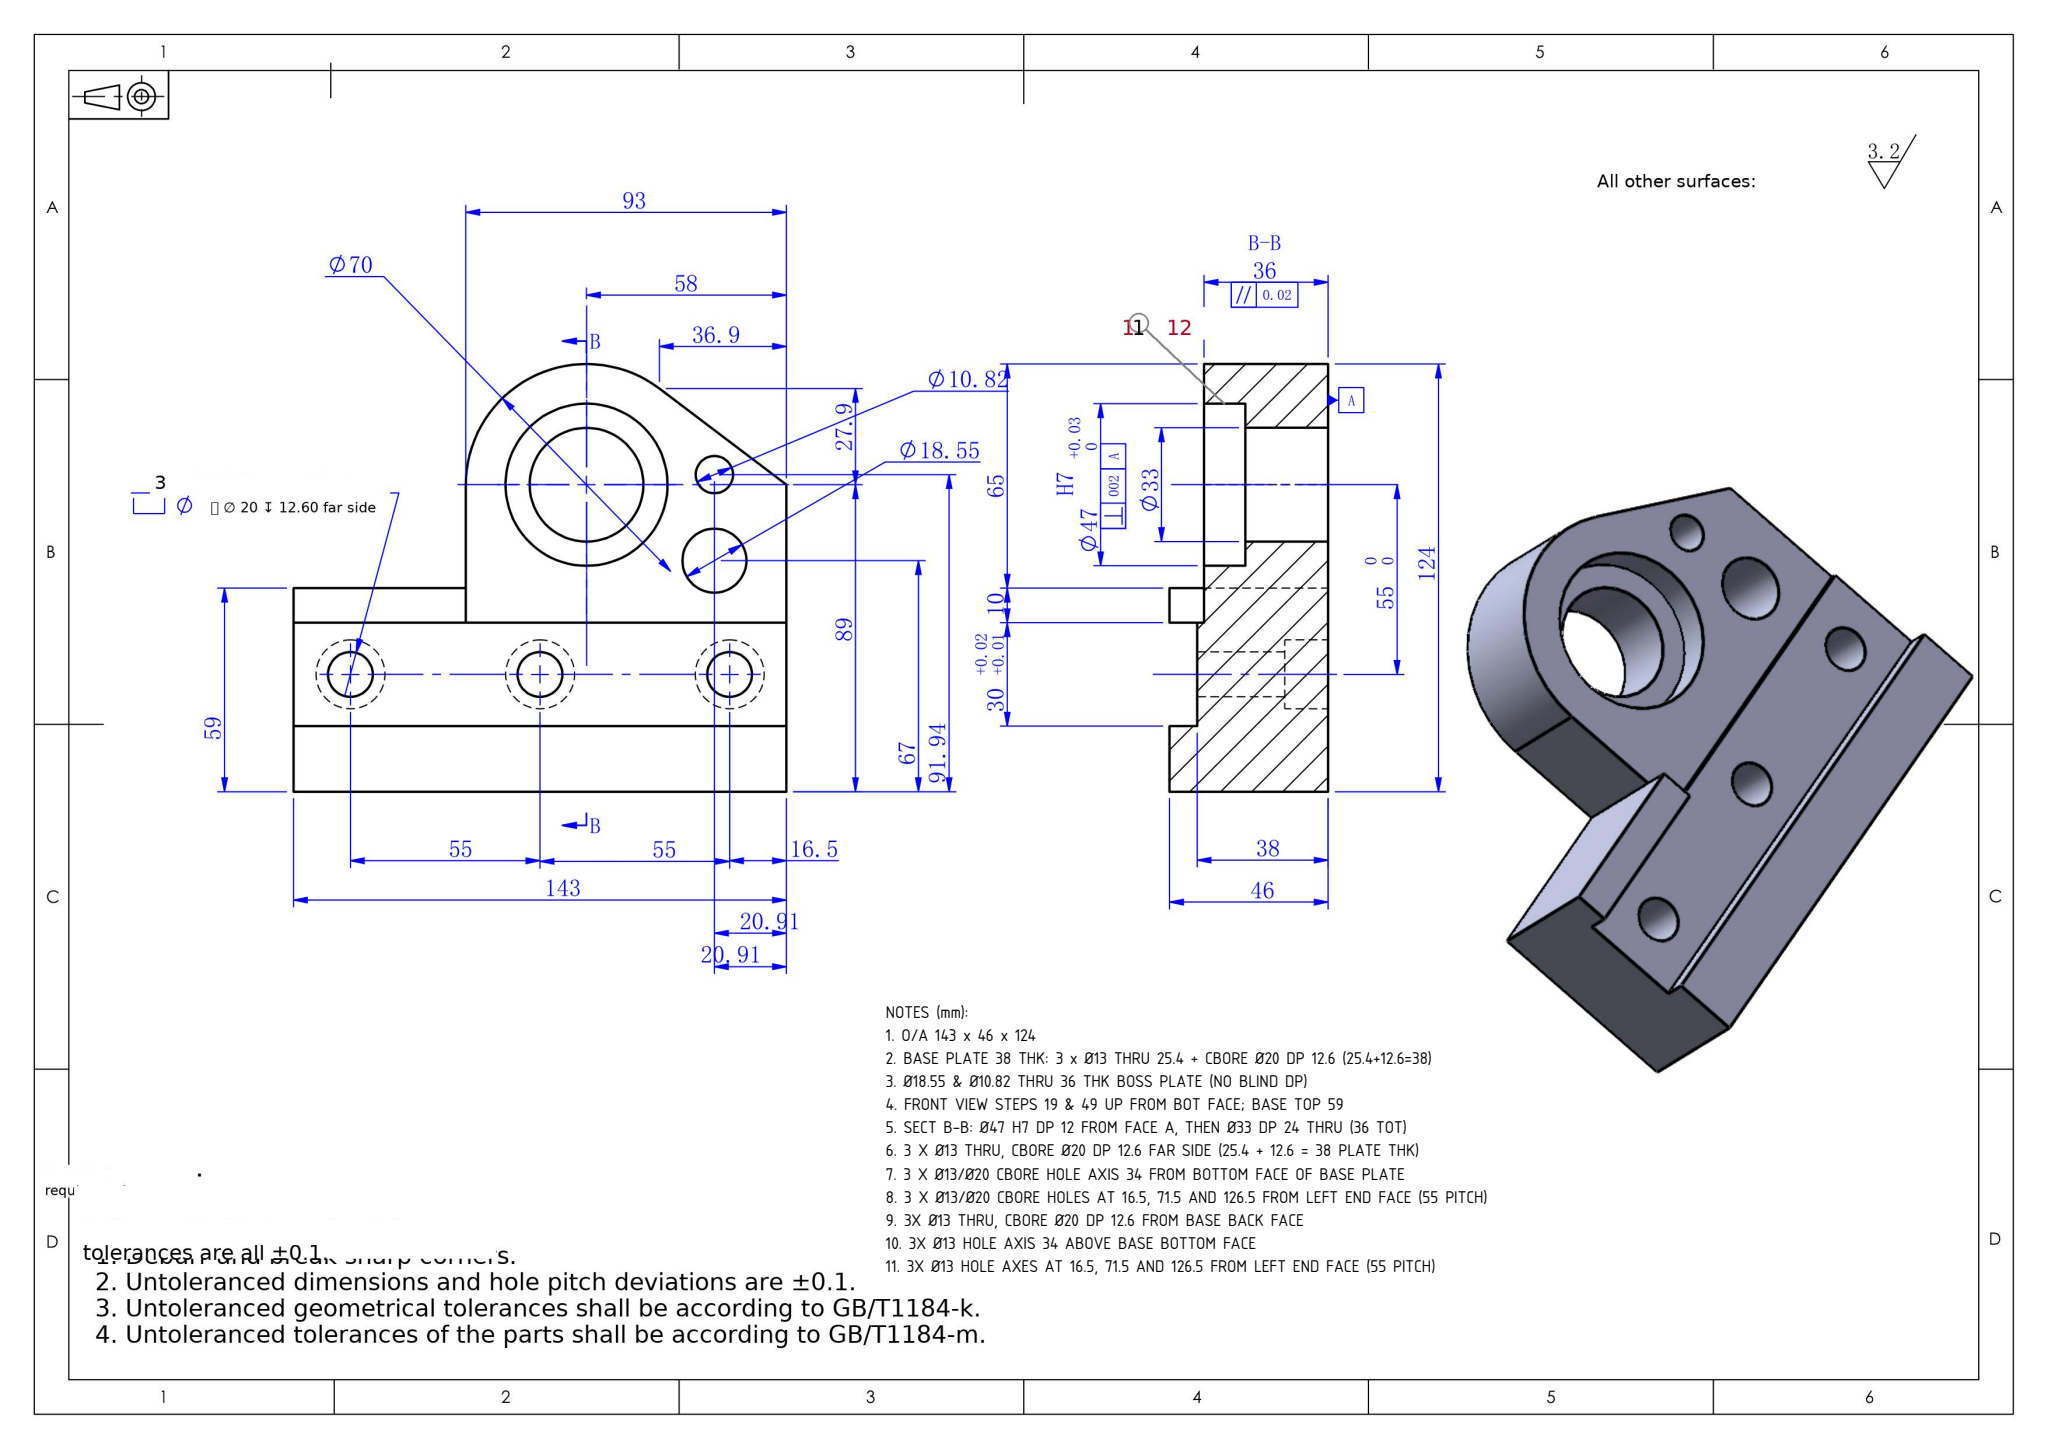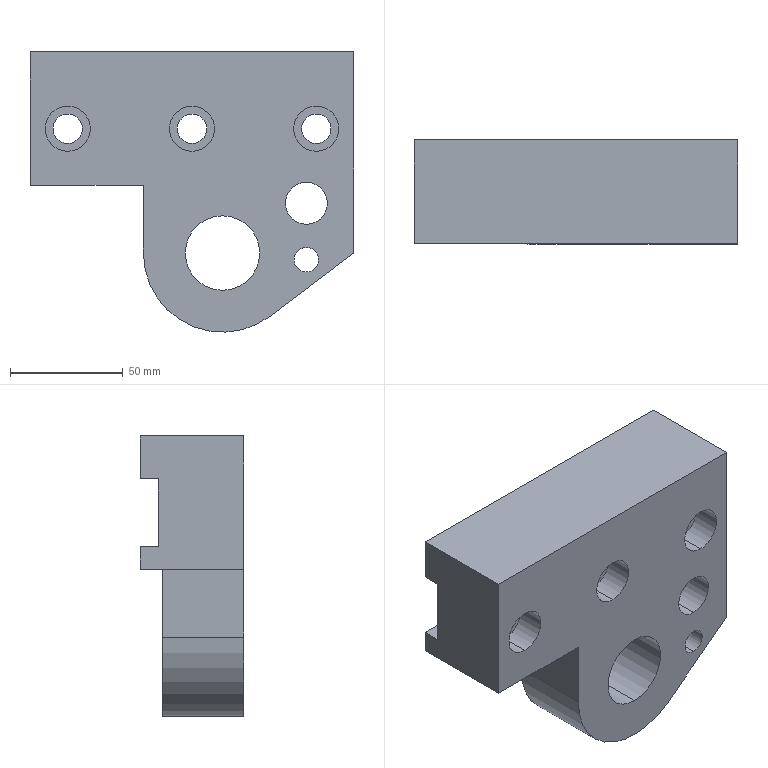Part | SolidWorks | mm | 1 solid | 40 faces | box 143 x 46 x 124 mm | volume 446604 mm3 | cylinder 21 | plane 19 | commonest cylinder face diameters 20 x6 13 x6 18.549 x2 10.821 x2 47 x2 33 x2 70 x1
Drawing notes:
O/A 143 x 46 x 124 | from the solid: bbox_xyz 143.0, 46.0, 124.0
BASE PLATE 38 THK: 3 x Ø13 THRU 25.4 + CBORE Ø20 DP 12.6 (25.4+12.6=38) | from the solid: y-planes 0,12.6(x3),38,46; Ø13 len 25.4 at x=16.5/71.5/126.5; Ø20 len 12.6
Ø18.55 & Ø10.82 THRU 36 THK BOSS PLATE (NO BLIND DP) | from the solid: cyl dia 18.549 & 10.821, axis y, len 36.0 = full boss plate y 0-36
FRONT VIEW STEPS 19 & 49 UP FROM BOT FACE; BASE TOP 59 | from the solid: z-planes 124,105,75,65 -> 19, 49, 59 above bottom face
SECT B-B: Ø47 H7 DP 12 FROM FACE A, THEN Ø33 DP 24 THRU (36 TOT) | from the solid: cylinders: [47.0,'y',[85,null,35],12.0] and [33.0,'y',[85,null,35],24.0]; boss thk 36 (y-planes 0..36)
3 X Ø13 THRU, CBORE Ø20 DP 12.6 FAR SIDE (25.4 + 12.6 = 38 PLATE THK) | from the solid: cylinders dia 13 len 25.4 and dia 20 len 12.6, axis y, at x = 16.5 / 71.5 / 126.5
3 X Ø13/Ø20 CBORE HOLE AXIS 34 FROM BOTTOM FACE OF BASE PLATE | from the solid: cylinders dia 13 and 20, axis y, z = 90 from bbox min; bbox z = 124, so 124 - 90 = 34 from bottom face
3 X Ø13/Ø20 CBORE HOLES AT 16.5, 71.5 AND 126.5 FROM LEFT END FACE (55 PITCH) | from the solid: cylinders dia 13 at x = 16.5, 71.5, 126.5; bbox x = 143
3X Ø13 THRU, CBORE Ø20 DP 12.6 FROM BASE BACK FACE | from the solid: cylinders dia 13 len 25.4 and dia 20 len 12.6 on axis y, same positions (16.5/71.5/126.5, z 90); y planes at 0, 12.6, 38
3X Ø13 HOLE AXIS 34 ABOVE BASE BOTTOM FACE | from the solid: dia 13 cylinders at z = 90 with bbox z = 124 (124 - 90 = 34 from bottom face)
3X Ø13 HOLE AXES AT 16.5, 71.5 AND 126.5 FROM LEFT END FACE (55 PITCH) | from the solid: dia 13 cylinder x positions 16.5, 71.5, 126.5 within bbox x = 143
build123d program:
from build123d import *

# Parameters (mm, degrees)
BOSS_EXTRUDE1_DEPTH                                  = 36
SKETCH2_W                                            = 49
SKETCH2_H                                            = 36
BOSS_EXTRUDE2_DEPTH                                  = 50
CYLINDRICAL_COUNTERSUNK_HOLE_FOR_M30_HEX_D           = 33
CYLINDRICAL_COUNTERSUNK_HOLE_FOR_M30_HEX_CBORE_D     = 47
CYLINDRICAL_COUNTERSUNK_HOLE_FOR_M30_HEX_CBORE_DEPTH = 12
SKETCH5_W                                            = 143
SKETCH5_H                                            = 19
BOSS_EXTRUDE3_DEPTH                                  = 10
SKETCH6_W                                            = 50
SKETCH6_H                                            = 46
BOSS_EXTRUDE4_DEPTH                                  = 10
SKETCH10_W                                           = 143
SKETCH10_H                                           = 30
BOSS_EXTRUDE5_DEPTH                                  = 2
M12_HEX_SOCKET_HEAD_CAP_SCREW_CBORE1_D               = 13
M12_HEX_SOCKET_HEAD_CAP_SCREW_CBORE1_CBORE_D         = 20
M12_HEX_SOCKET_HEAD_CAP_SCREW_CBORE1_CBORE_DEPTH     = 12.6
SKETCH11_R                                           = 9.275
SKETCH11_R_2                                         = 5.41
CUT_EXTRUDE1_DEPTH                                   = 96


with BuildPart() as part:
    # Sketch1 → Boss-Extrude1 (new body)
    with BuildSketch(Plane(origin=(0, -2704.978, 0), x_dir=(1, 0, 0), z_dir=(0, 1, 0))):
        with BuildLine():
            Line((-3455.015, -200.6), (-3455.015, -289.6))
            Line((-3455.015, -289.6), (-3362.015, -289.6))
            Line((-3362.015, -289.6), (-3362.015, -200.6))
            Line((-3362.015, -200.6), (-3398.894, -172.691))
            ThreePointArc((-3398.894, -172.691), (-3435.6, -169.261), (-3455.015, -200.6))
        make_face()
    extrude(amount=-BOSS_EXTRUDE1_DEPTH)

    # Sketch2 → Boss-Extrude2 (add)
    with BuildSketch(Plane.ZY.offset(3455.015)):
        with Locations((265.1, -2722.978)):
            Rectangle(SKETCH2_W, SKETCH2_H)
    extrude(amount=BOSS_EXTRUDE2_DEPTH)

    # Cylindrical Countersunk Hole for M30 Hex (through all)
    with Locations(Plane(origin=(0, -2704.978, 0), x_dir=(1, 0, 0), z_dir=(0, 1, 0))):
        with Locations((-3420.015, -200.6)):
            CounterBoreHole(CYLINDRICAL_COUNTERSUNK_HOLE_FOR_M30_HEX_D / 2, CYLINDRICAL_COUNTERSUNK_HOLE_FOR_M30_HEX_CBORE_D / 2, CYLINDRICAL_COUNTERSUNK_HOLE_FOR_M30_HEX_CBORE_DEPTH)

    # Sketch5 → Boss-Extrude3 (add)
    with BuildSketch(Plane(origin=(0, -2704.978, 0), x_dir=(1, 0, 0), z_dir=(0, 1, 0))):
        with Locations((-3433.515, -280.1)):
            Rectangle(SKETCH5_W, SKETCH5_H)
    extrude(amount=BOSS_EXTRUDE3_DEPTH)

    # Sketch6 → Boss-Extrude4 (add)
    with BuildSketch(Plane(origin=(0, 0, 240.6), x_dir=(-1, 0, 0), z_dir=(0, 0, -1))):
        with Locations((3480.015, -2717.978)):
            Rectangle(SKETCH6_W, SKETCH6_H)
    extrude(amount=BOSS_EXTRUDE4_DEPTH)

    # Sketch10 → Boss-Extrude5 (add)
    with BuildSketch(Plane(origin=(0, -2704.978, 0), x_dir=(1, 0, 0), z_dir=(0, 1, 0))):
        with Locations((-3433.515, -255.6)):
            Rectangle(SKETCH10_W, SKETCH10_H)
    extrude(amount=BOSS_EXTRUDE5_DEPTH)

    # M12 Hex Socket Head Cap Screw CBORE1 (through all)
    with Locations(Plane(origin=(0, -2740.978, 0), x_dir=(-1, 0, 0), z_dir=(0, -1, 0))):
        with Locations((3488.515, -255.6), (3433.515, -255.6), (3378.515, -255.6)):
            CounterBoreHole(M12_HEX_SOCKET_HEAD_CAP_SCREW_CBORE1_D / 2, M12_HEX_SOCKET_HEAD_CAP_SCREW_CBORE1_CBORE_D / 2, M12_HEX_SOCKET_HEAD_CAP_SCREW_CBORE1_CBORE_DEPTH)

    # Sketch11 → Cut-Extrude1 (cut)
    with BuildSketch(Plane(origin=(0, -2704.978, 0), x_dir=(1, 0, 0), z_dir=(0, 1, 0))):
        with Locations(Location((-3382.924, -222.601, 0), (0, 0, 270))):
            Circle(SKETCH11_R)
        with Locations(Location((-3382.924, -197.665, 0), (0, 0, 270))):
            Circle(SKETCH11_R_2)
    extrude(amount=-CUT_EXTRUDE1_DEPTH, mode=Mode.SUBTRACT)


solid = part.part